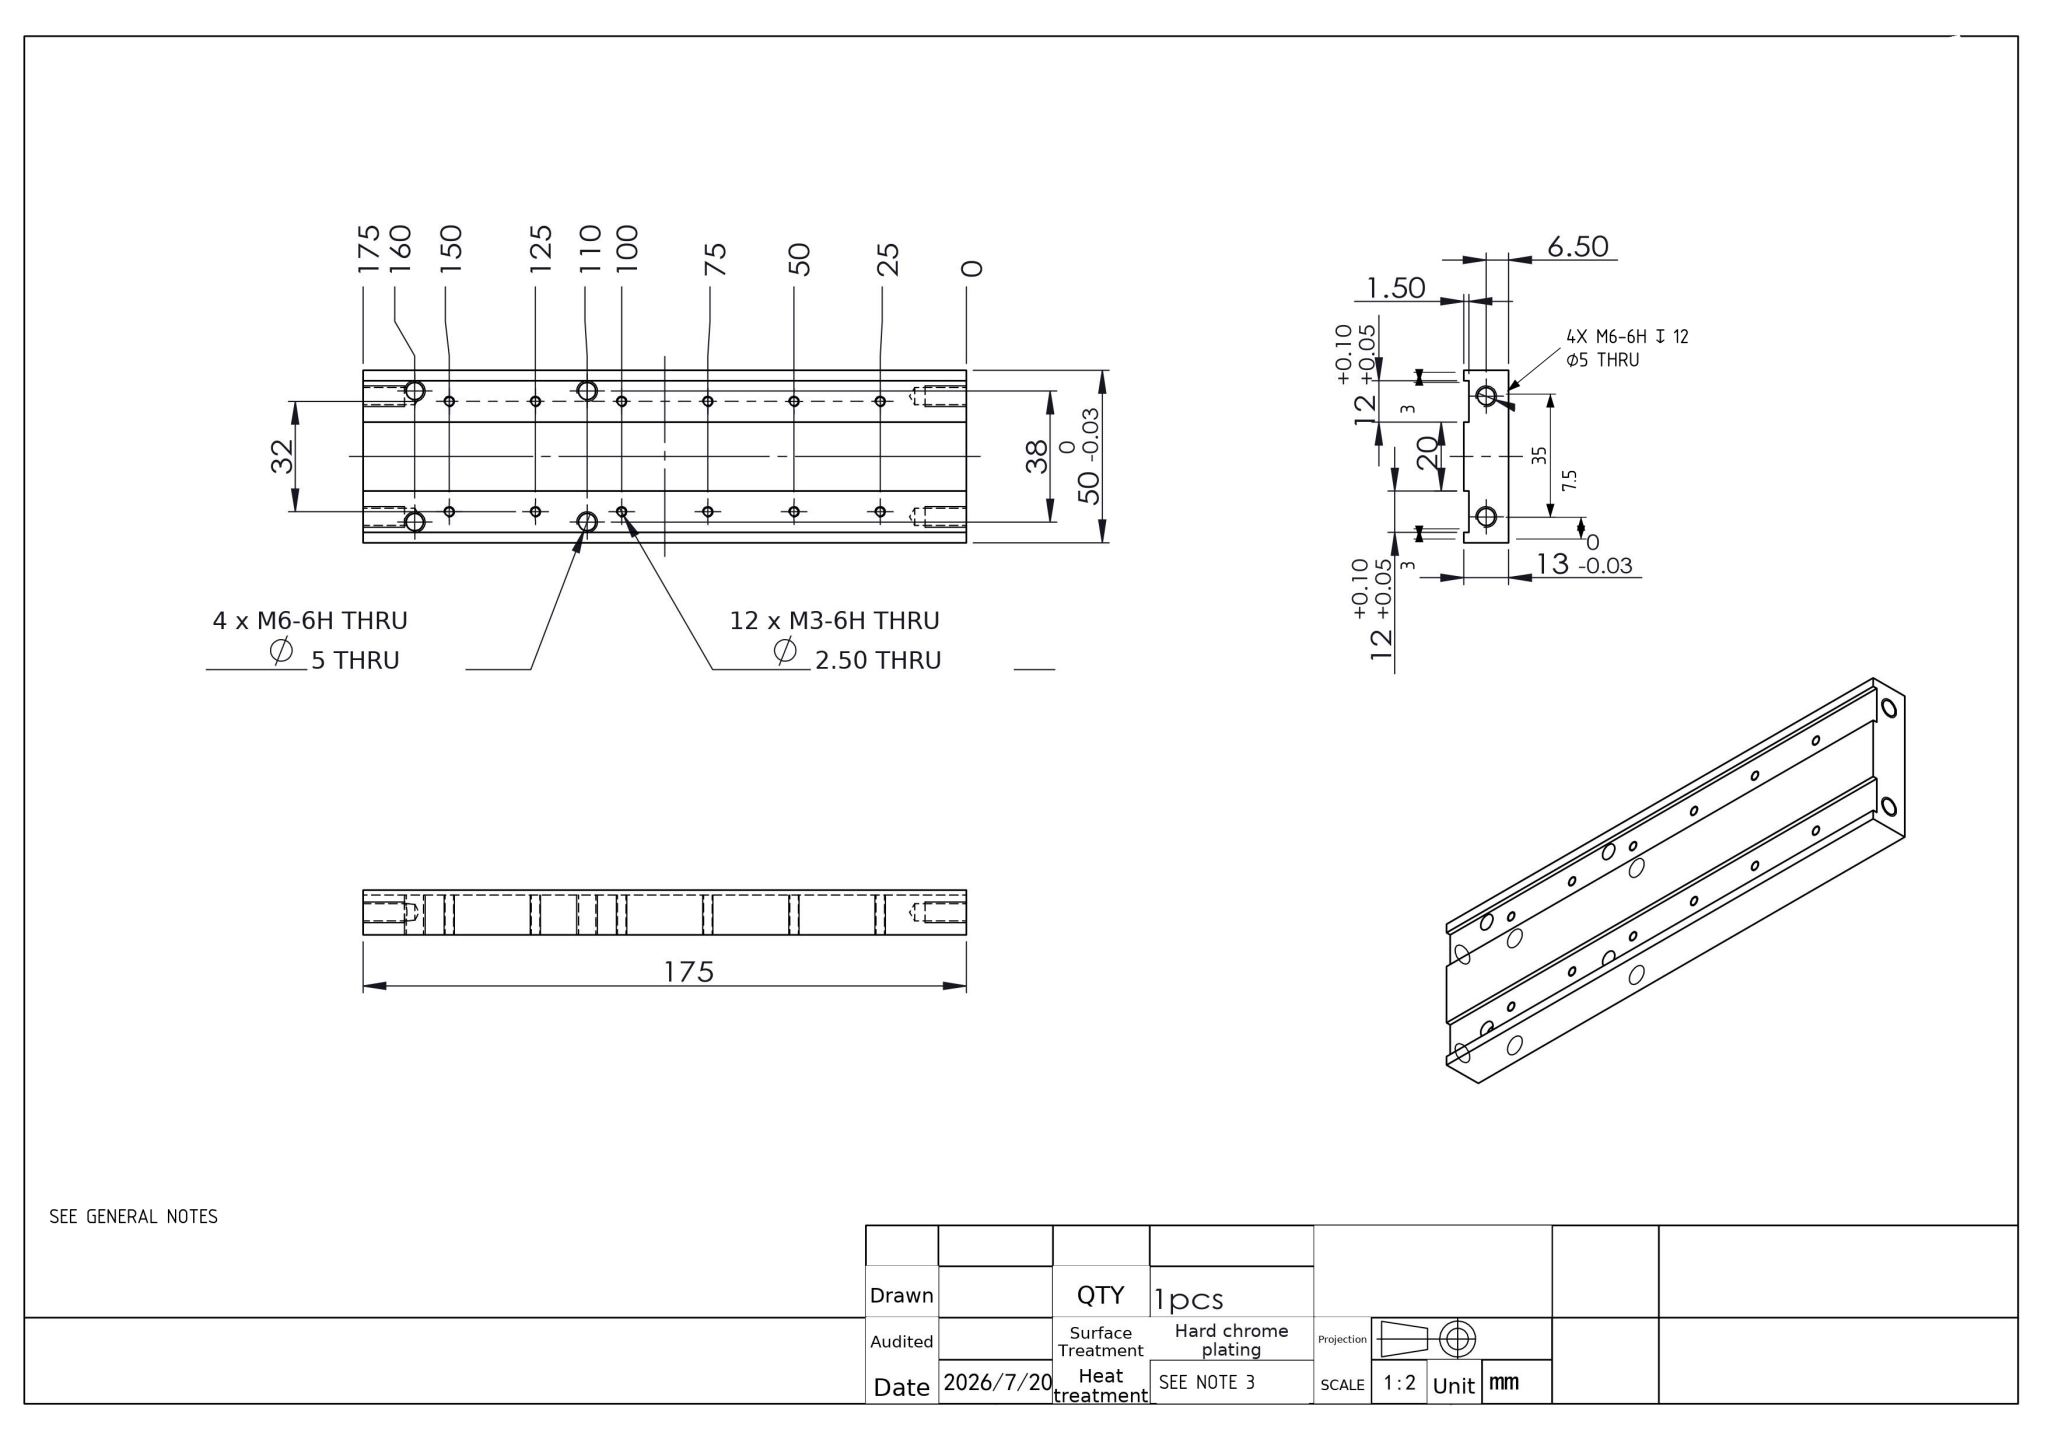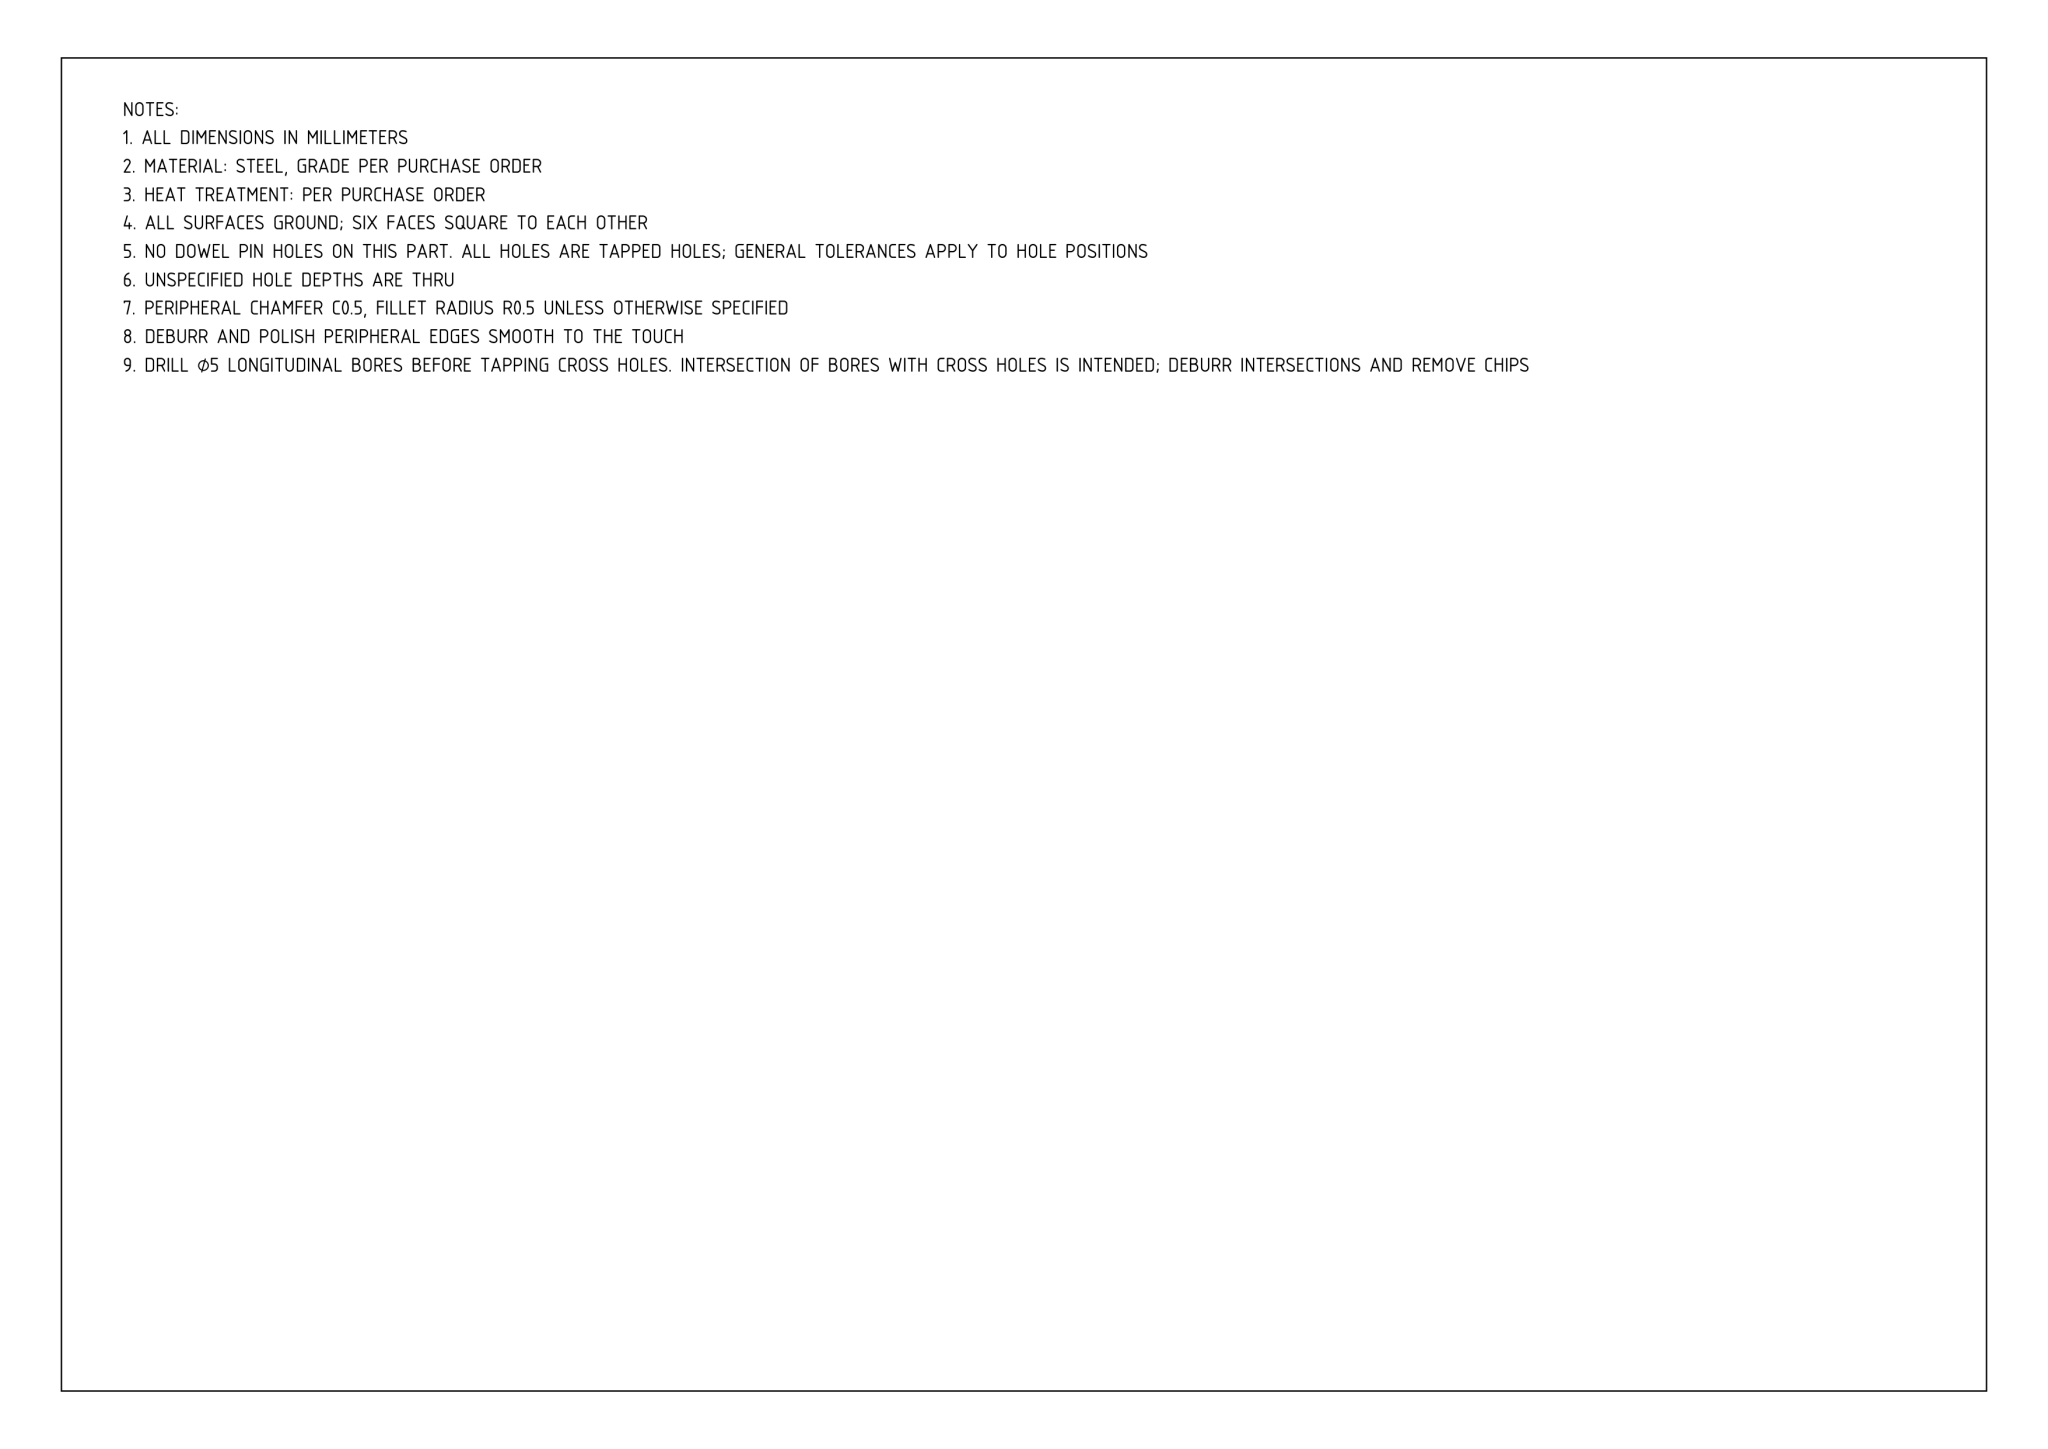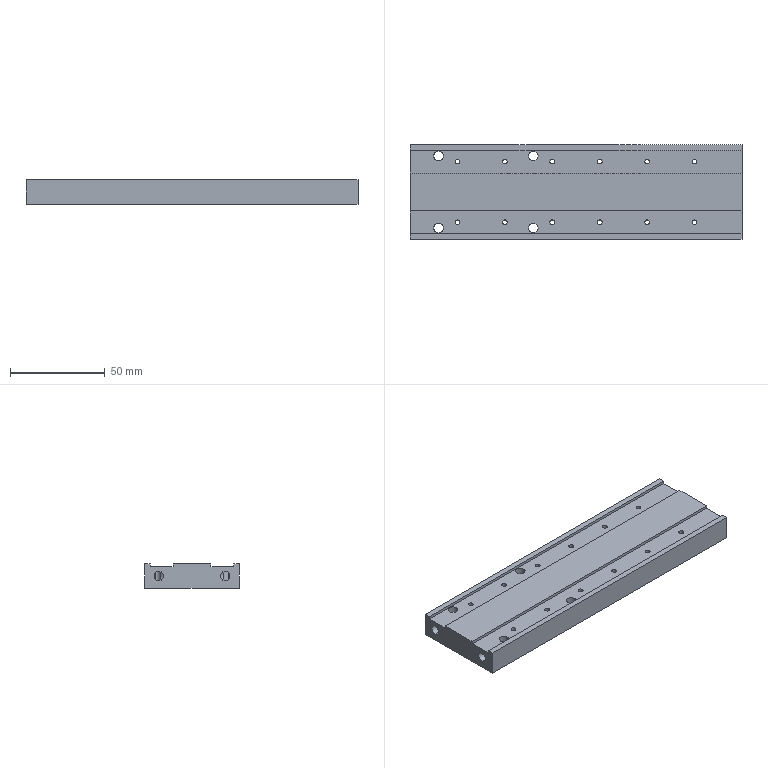Part | NX | mm | 1 solid | 60 faces | box 175 x 50 x 13 mm | volume 104728 mm3 | cylinder 40 | plane 14 | cone 6 | commonest cylinder face diameters 2.5 x24 5 x16